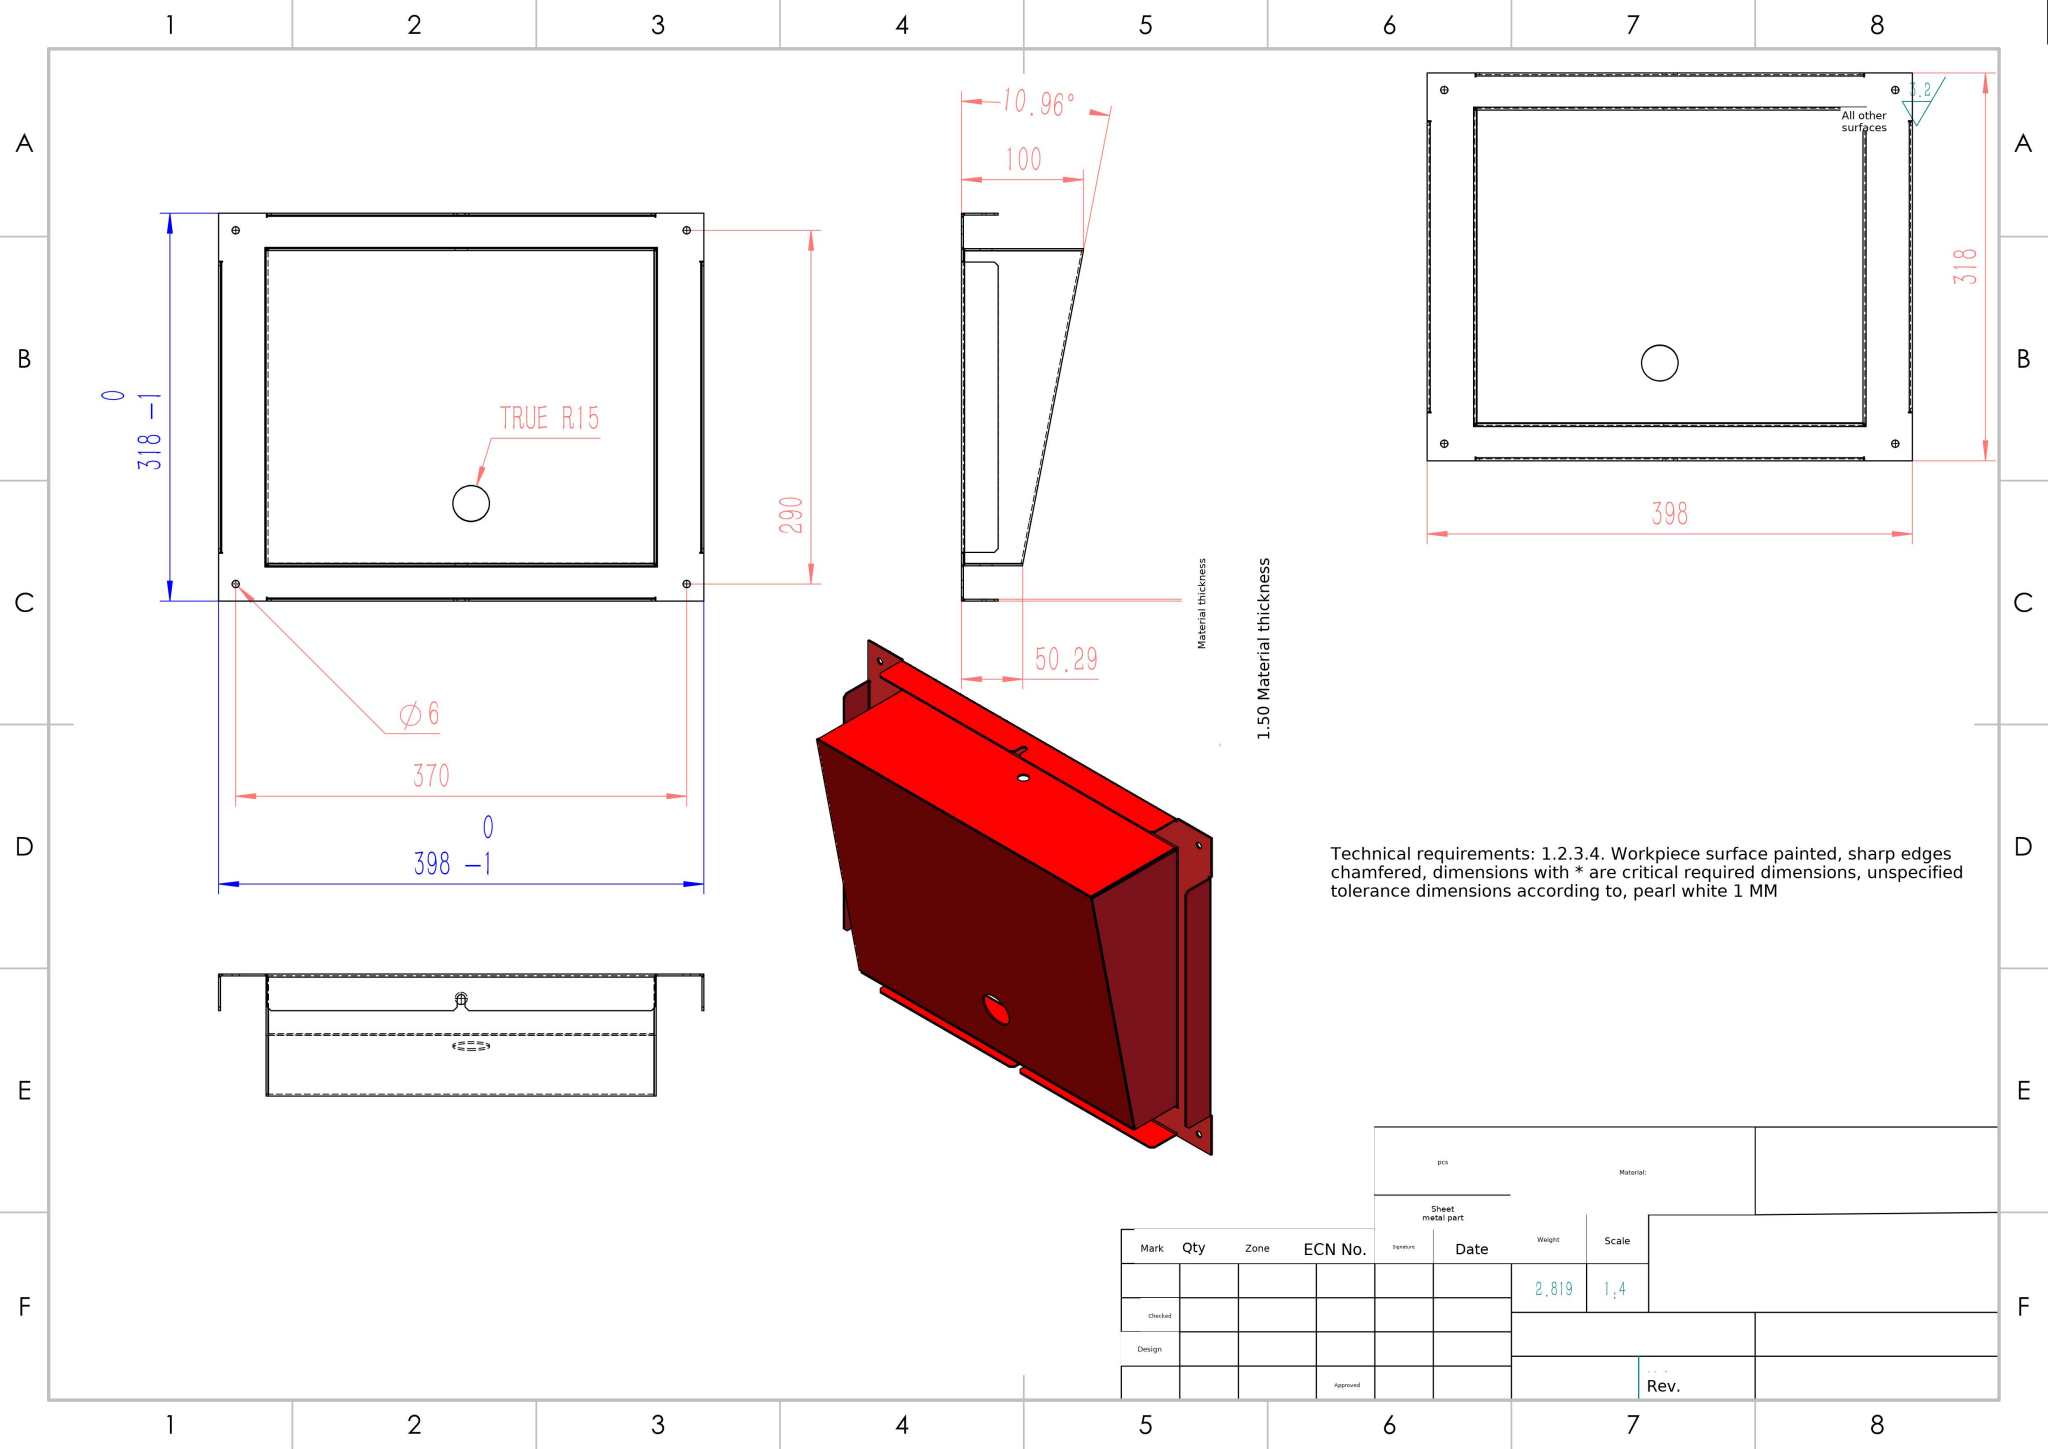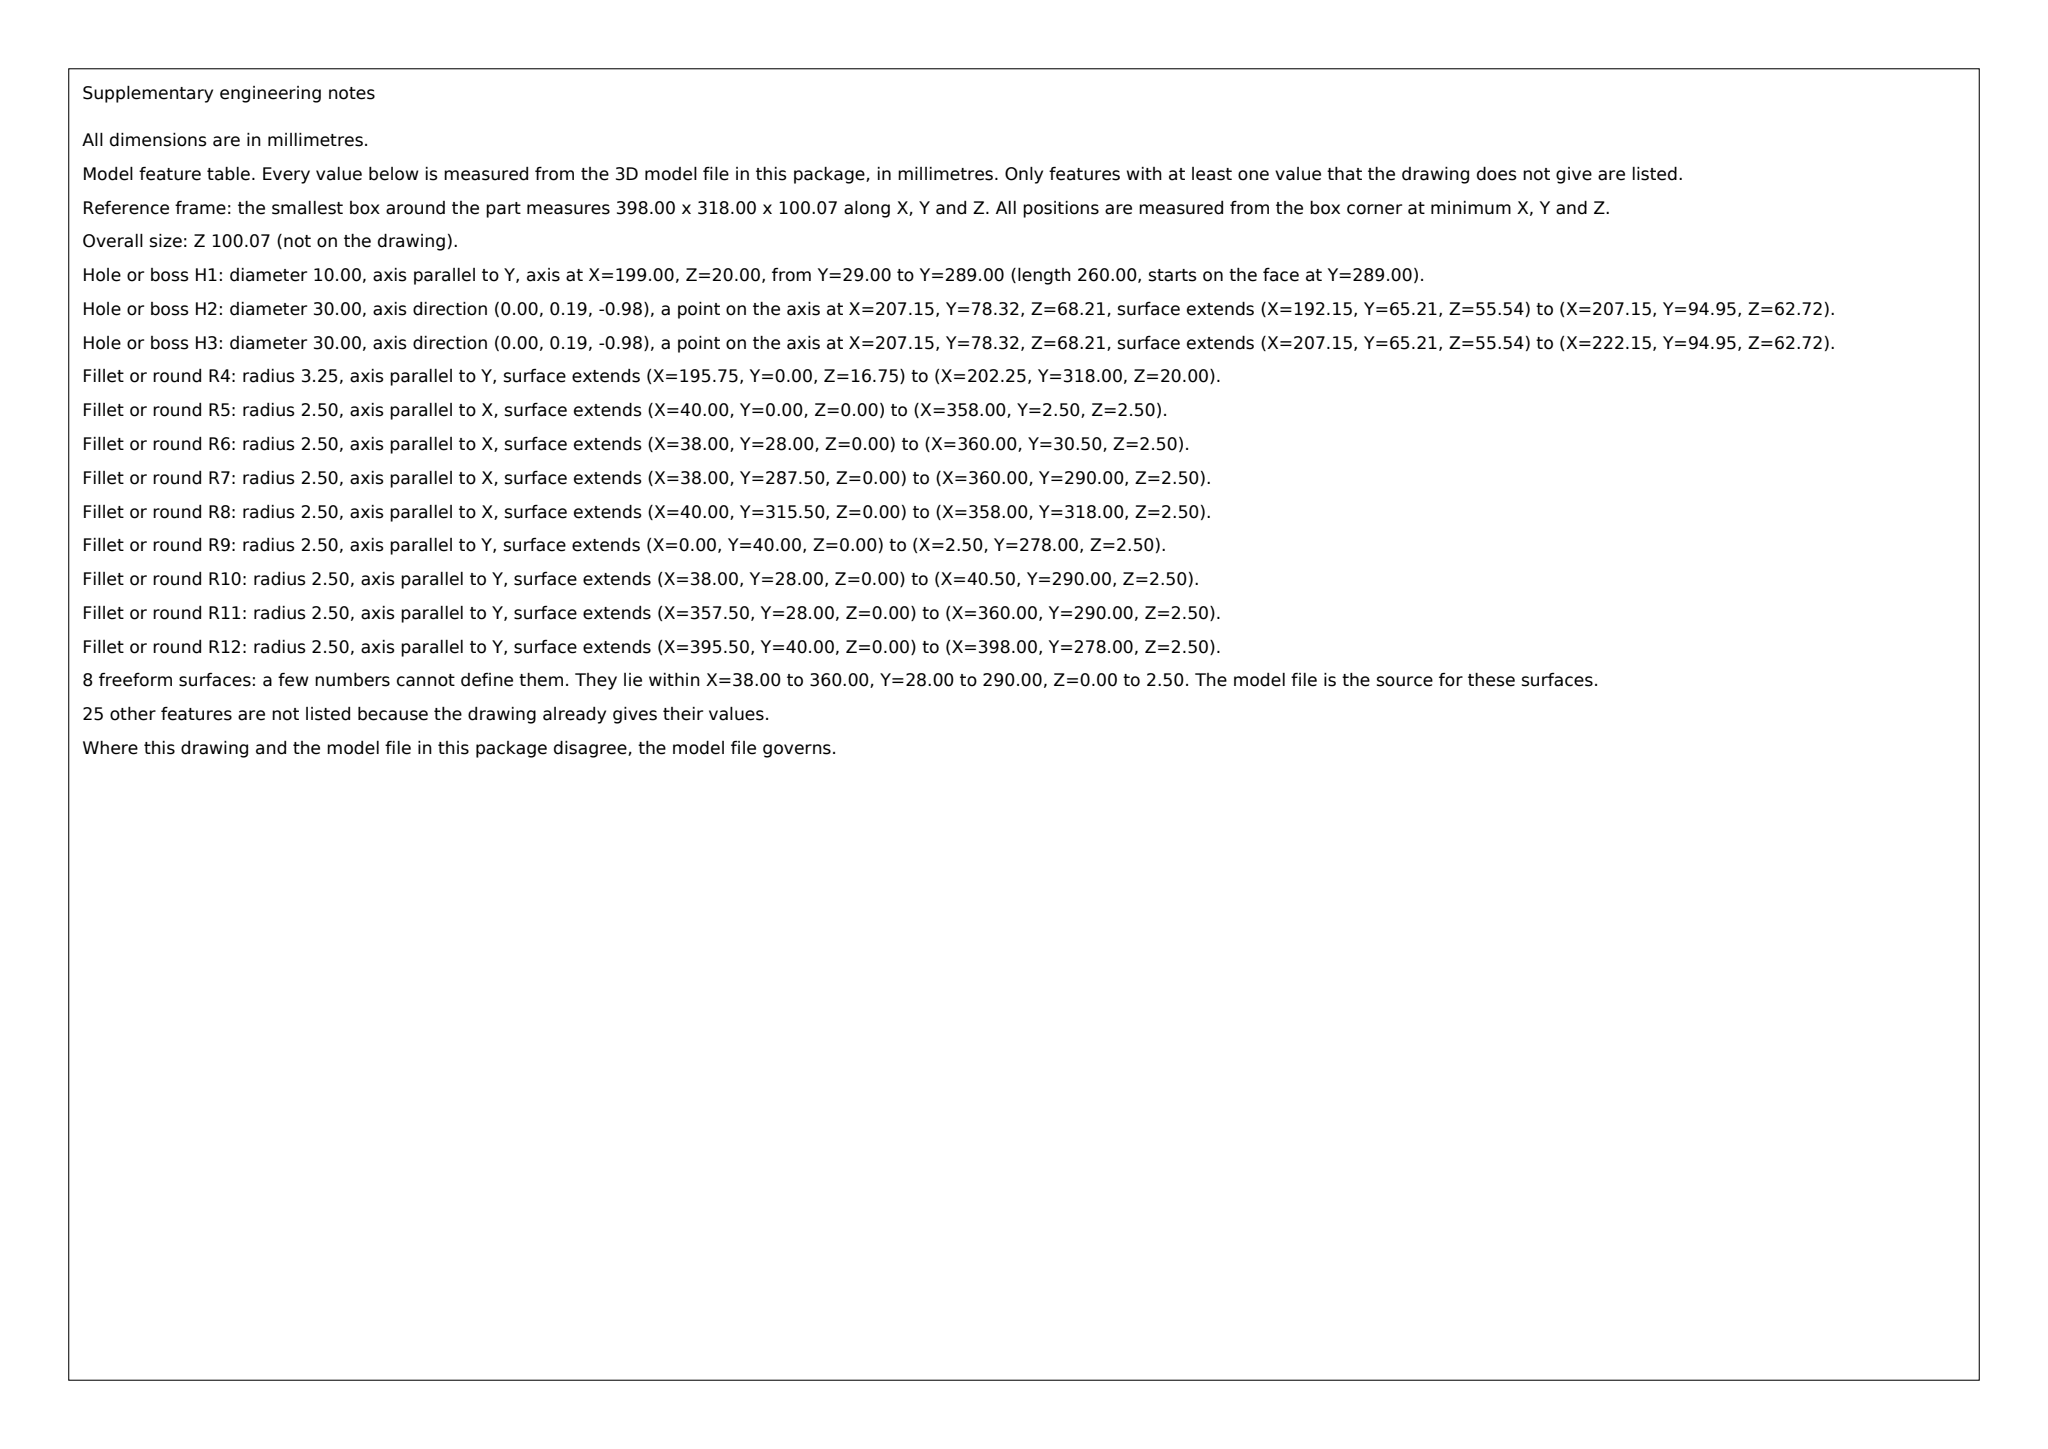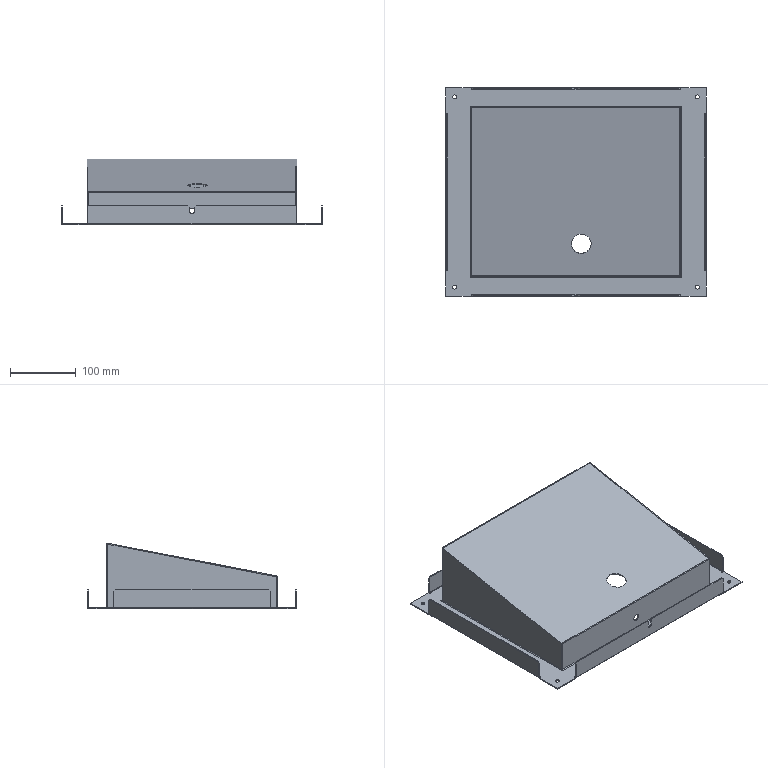Part | SolidWorks | mm | 1 solid | 143 faces | box 398 x 318 x 100.07 mm | volume 361418 mm3 | plane 103 | cylinder 32 | spline 8 | commonest cylinder face diameters 6 x8 5 x8 2 x8 10 x4 30 x2 6.5 x2